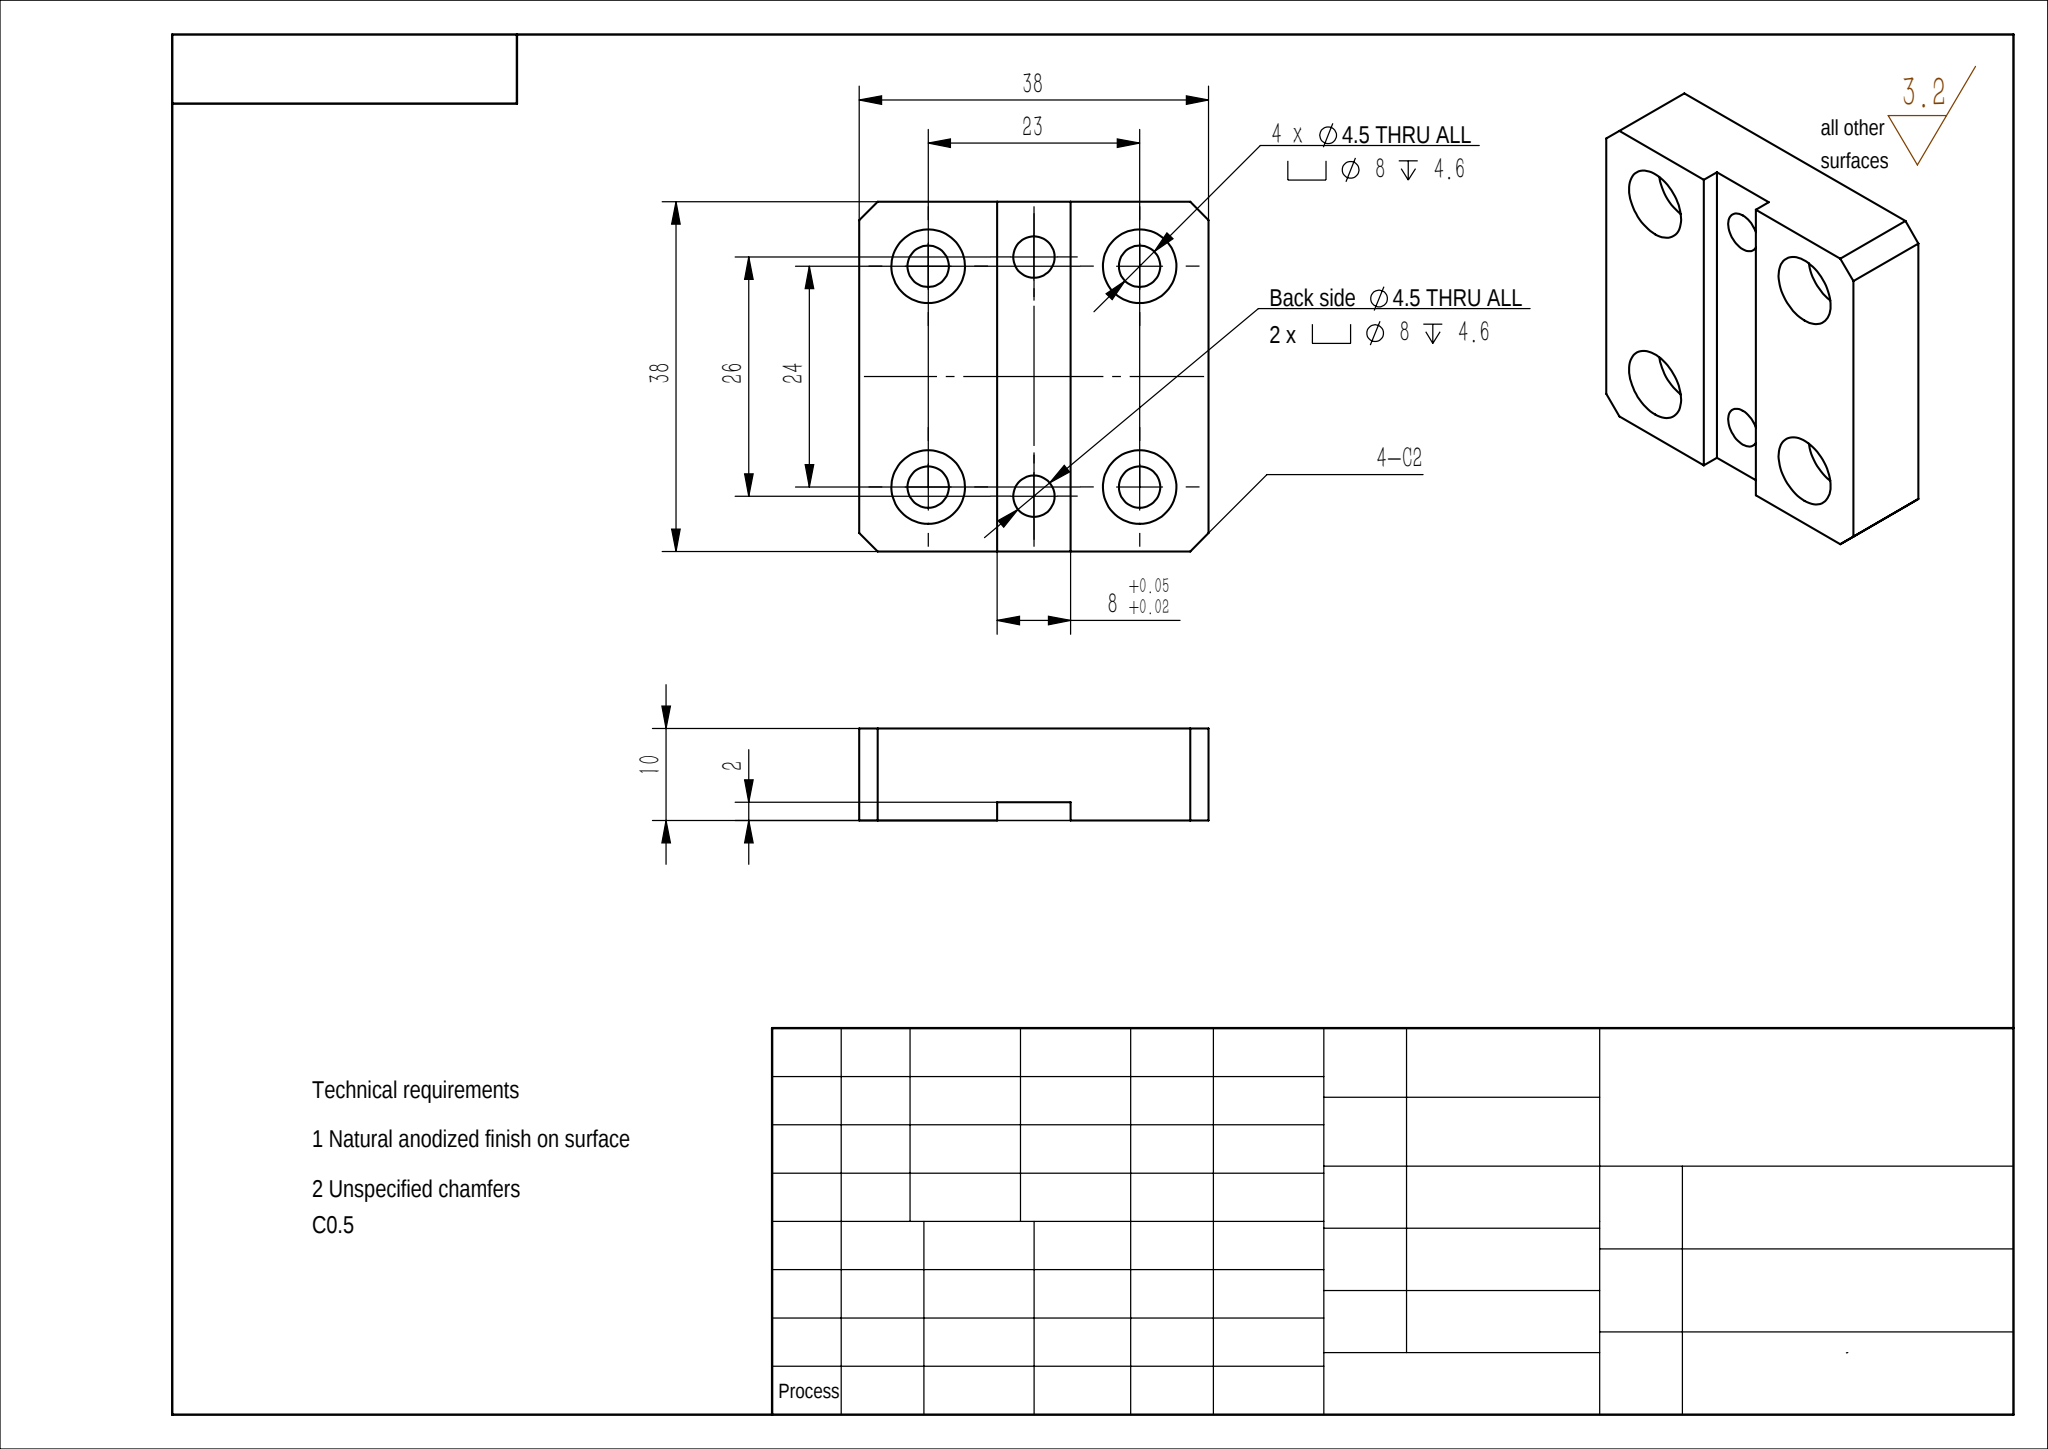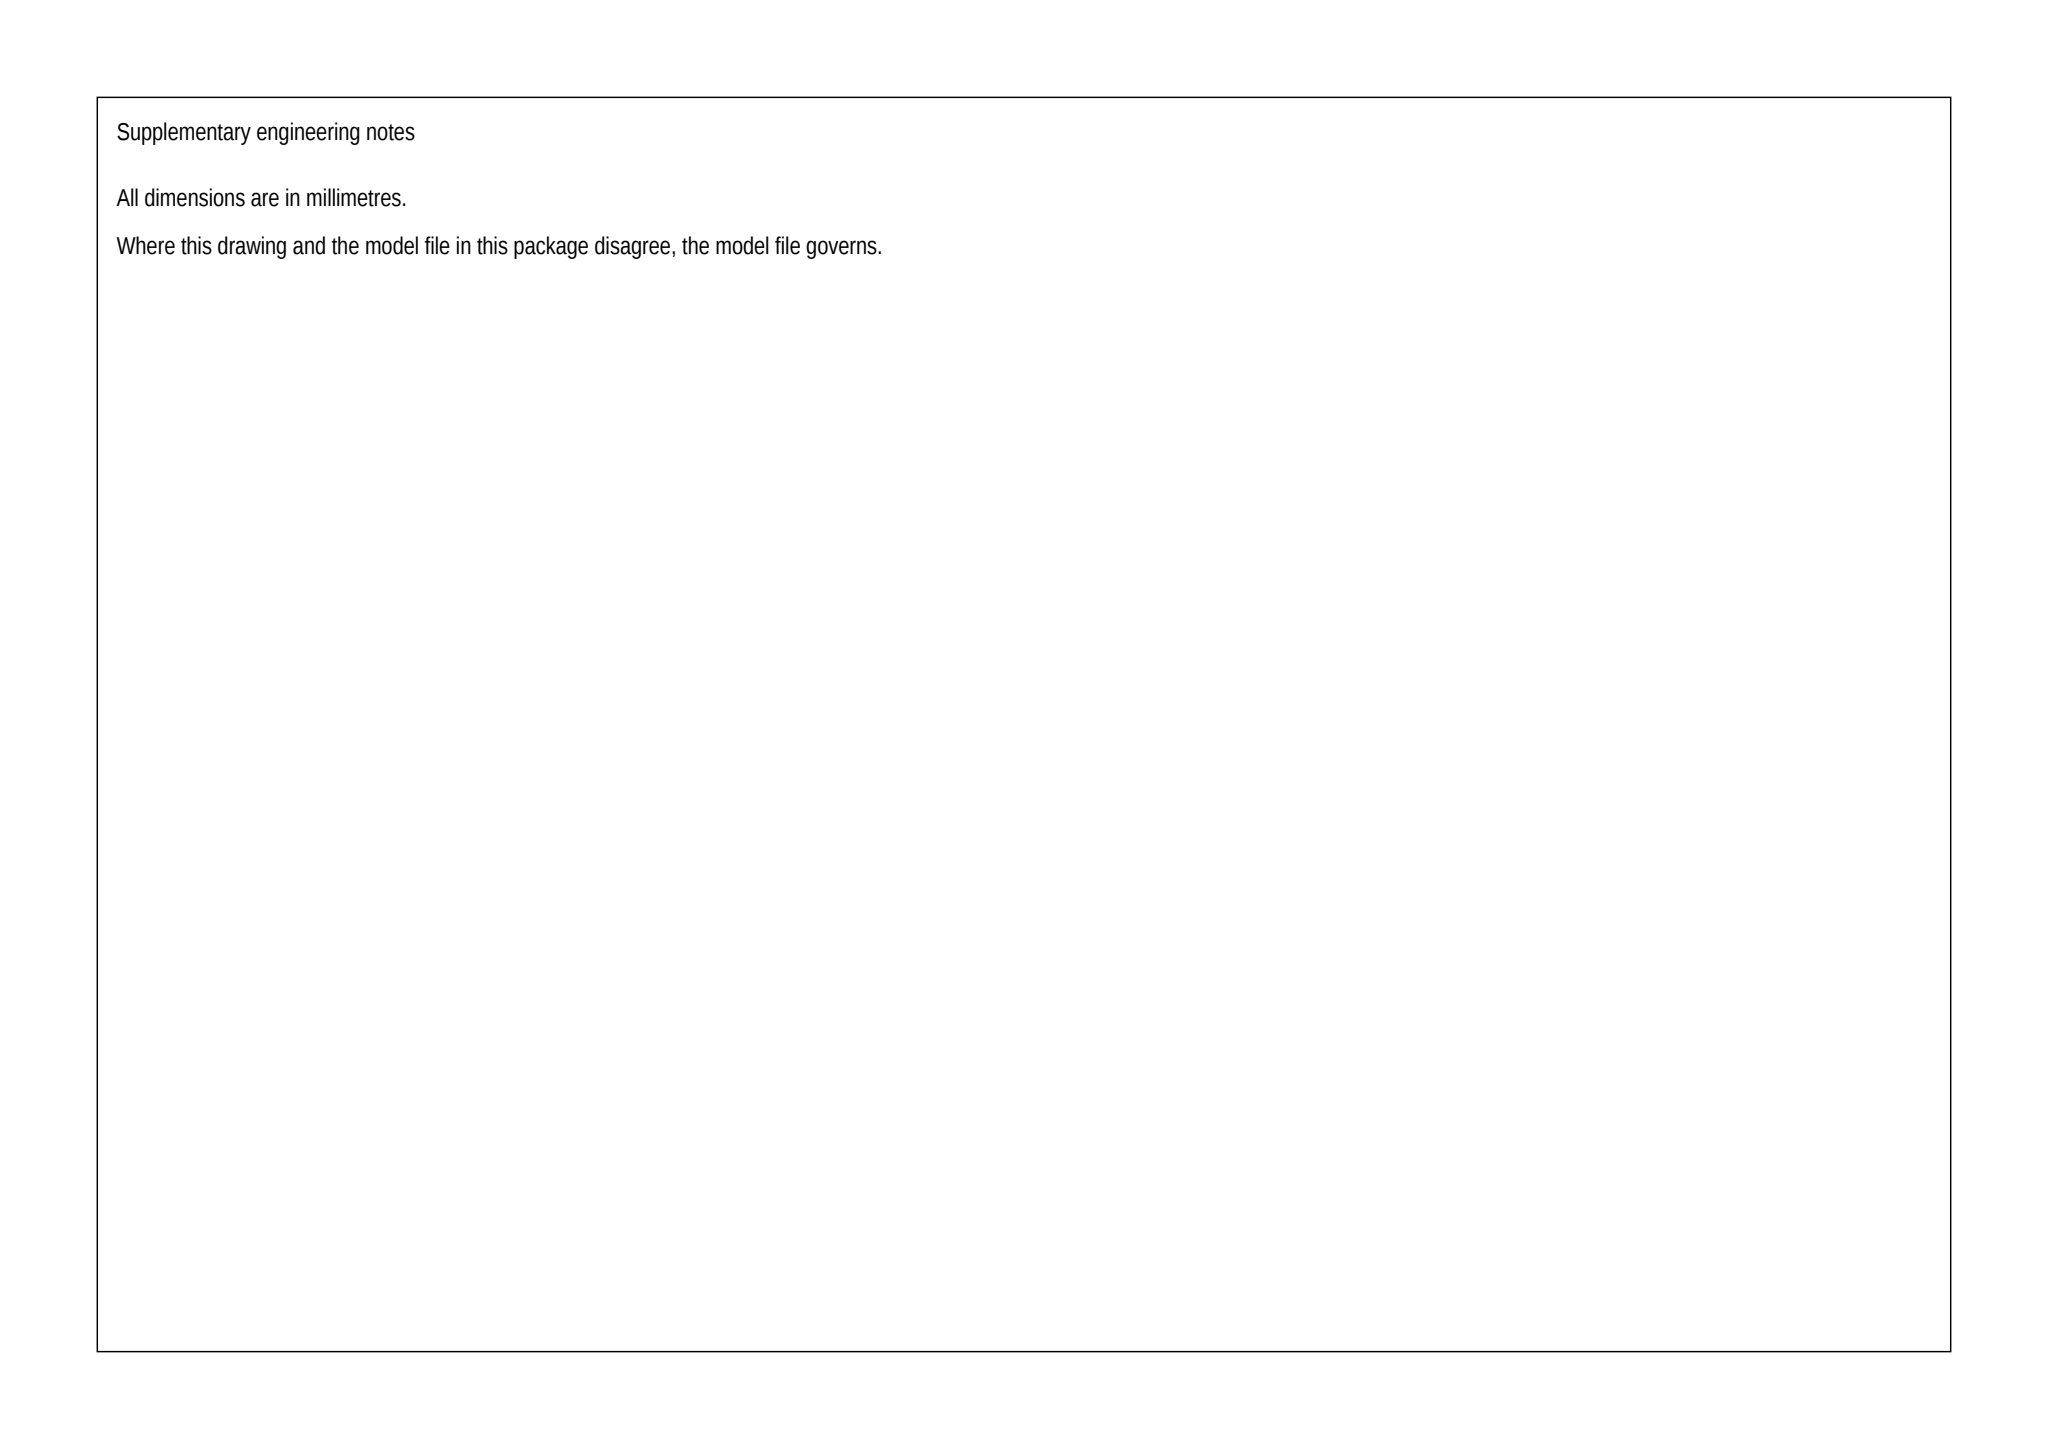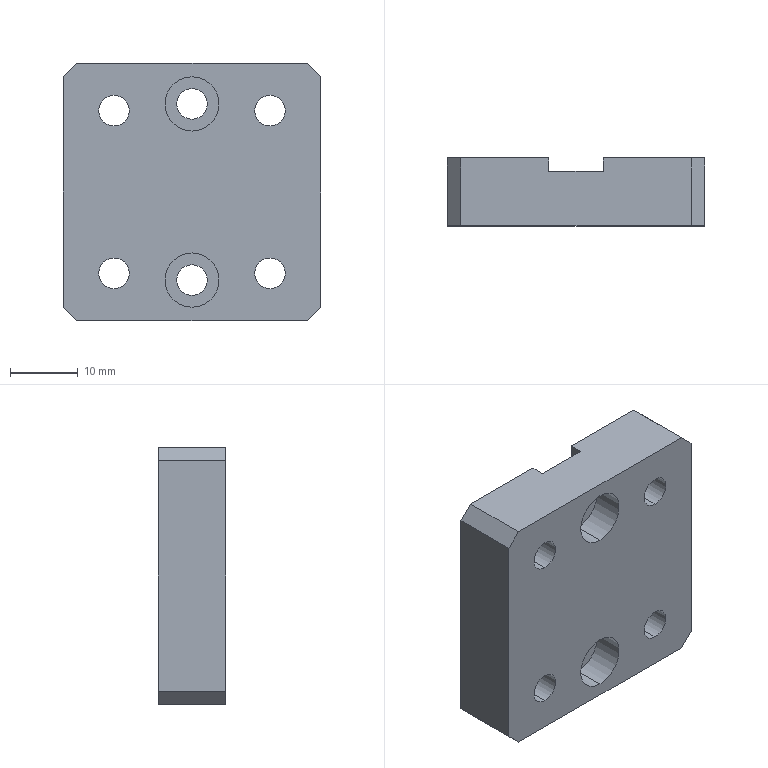Part | SolidWorks | mm | 1 solid | 44 faces | box 38 x 10 x 38 mm | volume 11913 mm3 | cylinder 24 | plane 20 | commonest cylinder face diameters 8 x12 4.5 x12
Drawing notes:
8 +0.05/+0.02 SLOT CL ON 38 CL; WALL FACE 15 FROM LH EDGE | from the solid: x-planes at 15.0 and 23.0 in 38.0 wide bbox => slot centered at x=19
HOLE COLS 7.5 & 30.5 FROM LH EDGE; CTR COL 19 = 38 CL | from the solid: Ø4.5 axes at x=7.5, 19.0, 30.5 (23 between outer cols)
4X Ø8 DP 4.6 CBORE FROM FRONT FACE; 2X Ø8 DP 4.6 FROM BACK FACE | from the solid: CB floors y=5.4 (4 holes, x=7.5/30.5, entered y=10); y=4.6 (2 holes, x=19, entered y=0)
2 DEEP RECESS CUT FROM FRONT FACE; FLOOR 8 FROM BACK FACE | from the solid: y-plane 8.0 recess floor, bbox y=10, outer faces at y=10
build123d program:
from build123d import *

# Parameters (mm, degrees)
SKETCH1_W                                         = 38
SKETCH1_H                                         = 38
BOSS_EXTRUDE1_DEPTH                               = 10
SKETCH2_W                                         = 8
SKETCH2_H                                         = 52.789
CUT_EXTRUDE1_DEPTH                                = 2
HOLE_SIZE_ACCORDING_TO_HEXAGON_SOCKET_D           = 4.5
HOLE_SIZE_ACCORDING_TO_HEXAGON_SOCKET_CBORE_D     = 8
HOLE_SIZE_ACCORDING_TO_HEXAGON_SOCKET_CBORE_DEPTH = 4.6
HOLE_SIZE_ACCORDING_TO_HEXAGON_SO_2_D             = 4.5
HOLE_SIZE_ACCORDING_TO_HEXAGON_SO_2_CBORE_D       = 8
HOLE_SIZE_ACCORDING_TO_HEXAGON_SO_2_CBORE_DEPTH   = 4.6
CHAMFER1_SIZE                                     = 2


with BuildPart() as part:
    # Sketch1 → Boss-Extrude1 (new body)
    with BuildSketch(Plane(origin=(0, 0, 0), x_dir=(1, 0, 0), z_dir=(0, 1, 0))):
        Rectangle(SKETCH1_W, SKETCH1_H)
    extrude(amount=BOSS_EXTRUDE1_DEPTH)

    # Sketch2 → Cut-Extrude1 (cut)
    with BuildSketch(Plane(origin=(0, 10, 0), x_dir=(1, 0, 0), z_dir=(0, 1, 0))):
        Rectangle(SKETCH2_W, SKETCH2_H)
    extrude(amount=-CUT_EXTRUDE1_DEPTH, mode=Mode.SUBTRACT)

    # Hole Size _ according to_ Hexagon Socket (through all)
    with Locations(Plane(origin=(0, 10, 0), x_dir=(1, 0, 0), z_dir=(0, 1, 0))):
        with Locations((-11.5, 12), (-11.5, -12), (11.5, 12), (11.5, -12)):
            CounterBoreHole(HOLE_SIZE_ACCORDING_TO_HEXAGON_SOCKET_D / 2, HOLE_SIZE_ACCORDING_TO_HEXAGON_SOCKET_CBORE_D / 2, HOLE_SIZE_ACCORDING_TO_HEXAGON_SOCKET_CBORE_DEPTH)

    # Hole Size _ according to_ Hexagon So 2 (through all)
    with Locations(Plane(origin=(0, 0, 0), x_dir=(-1, 0, 0), z_dir=(0, -1, 0))):
        with Locations((0, -13), (0, 13)):
            CounterBoreHole(HOLE_SIZE_ACCORDING_TO_HEXAGON_SO_2_D / 2, HOLE_SIZE_ACCORDING_TO_HEXAGON_SO_2_CBORE_D / 2, HOLE_SIZE_ACCORDING_TO_HEXAGON_SO_2_CBORE_DEPTH)

    # Chamfer1
    chamfer1_edges = [part.edges().sort_by_distance(p)[0] for p in [
        (19, 5, 19),
        (-19, 5, 19),
        (-19, 5, -19),
        (19, 5, -19),
    ]]
    chamfer(chamfer1_edges, length=CHAMFER1_SIZE)


solid = part.part